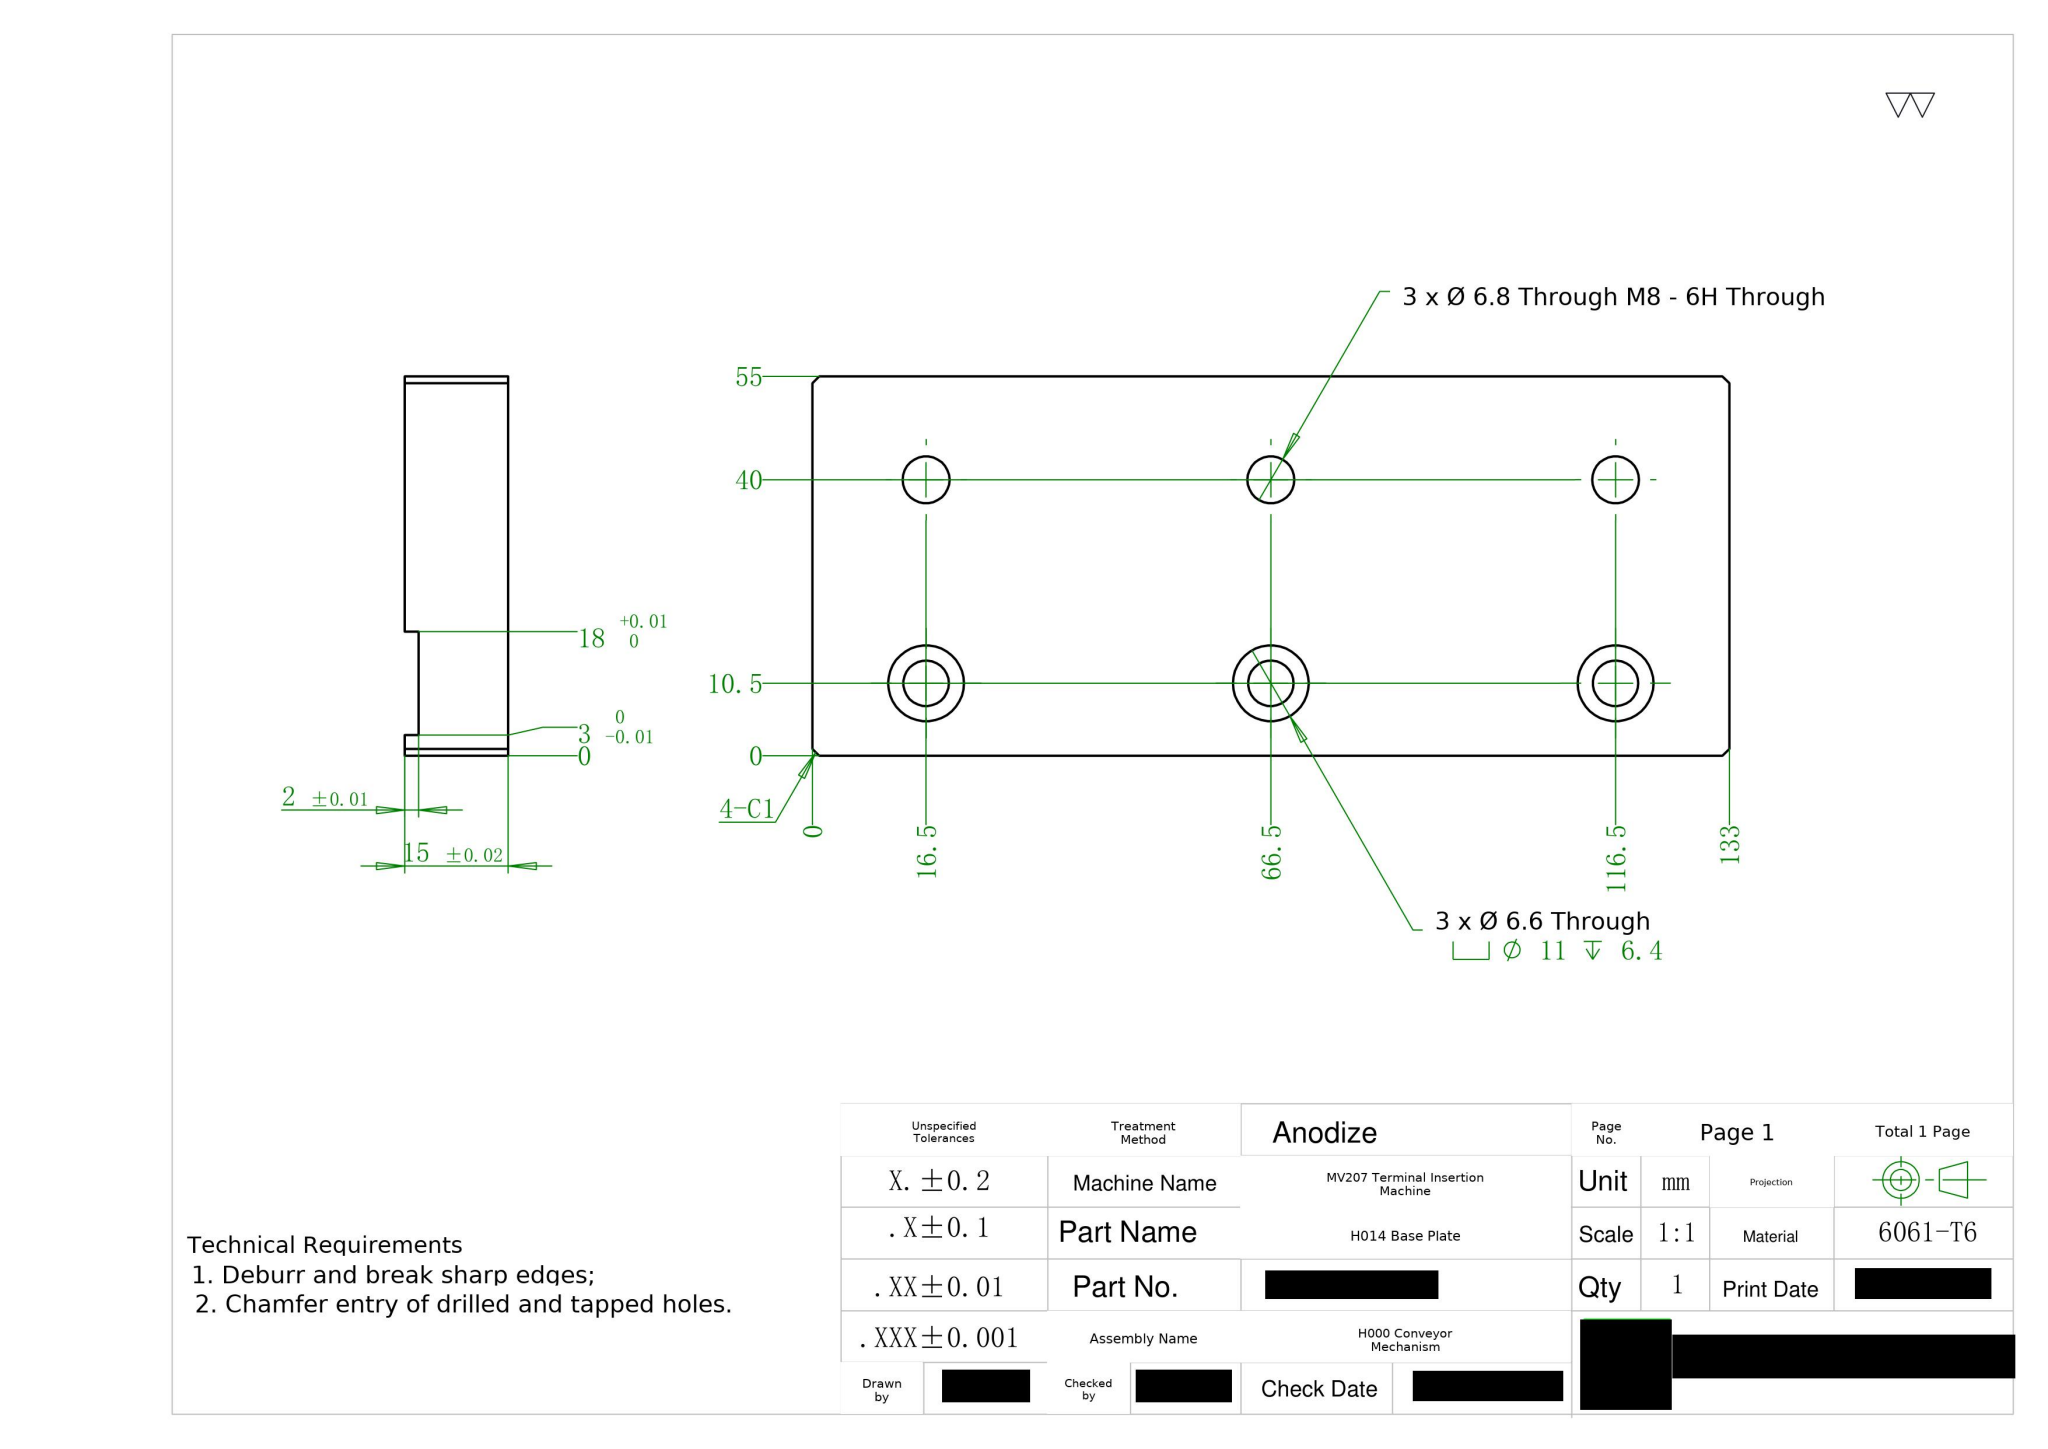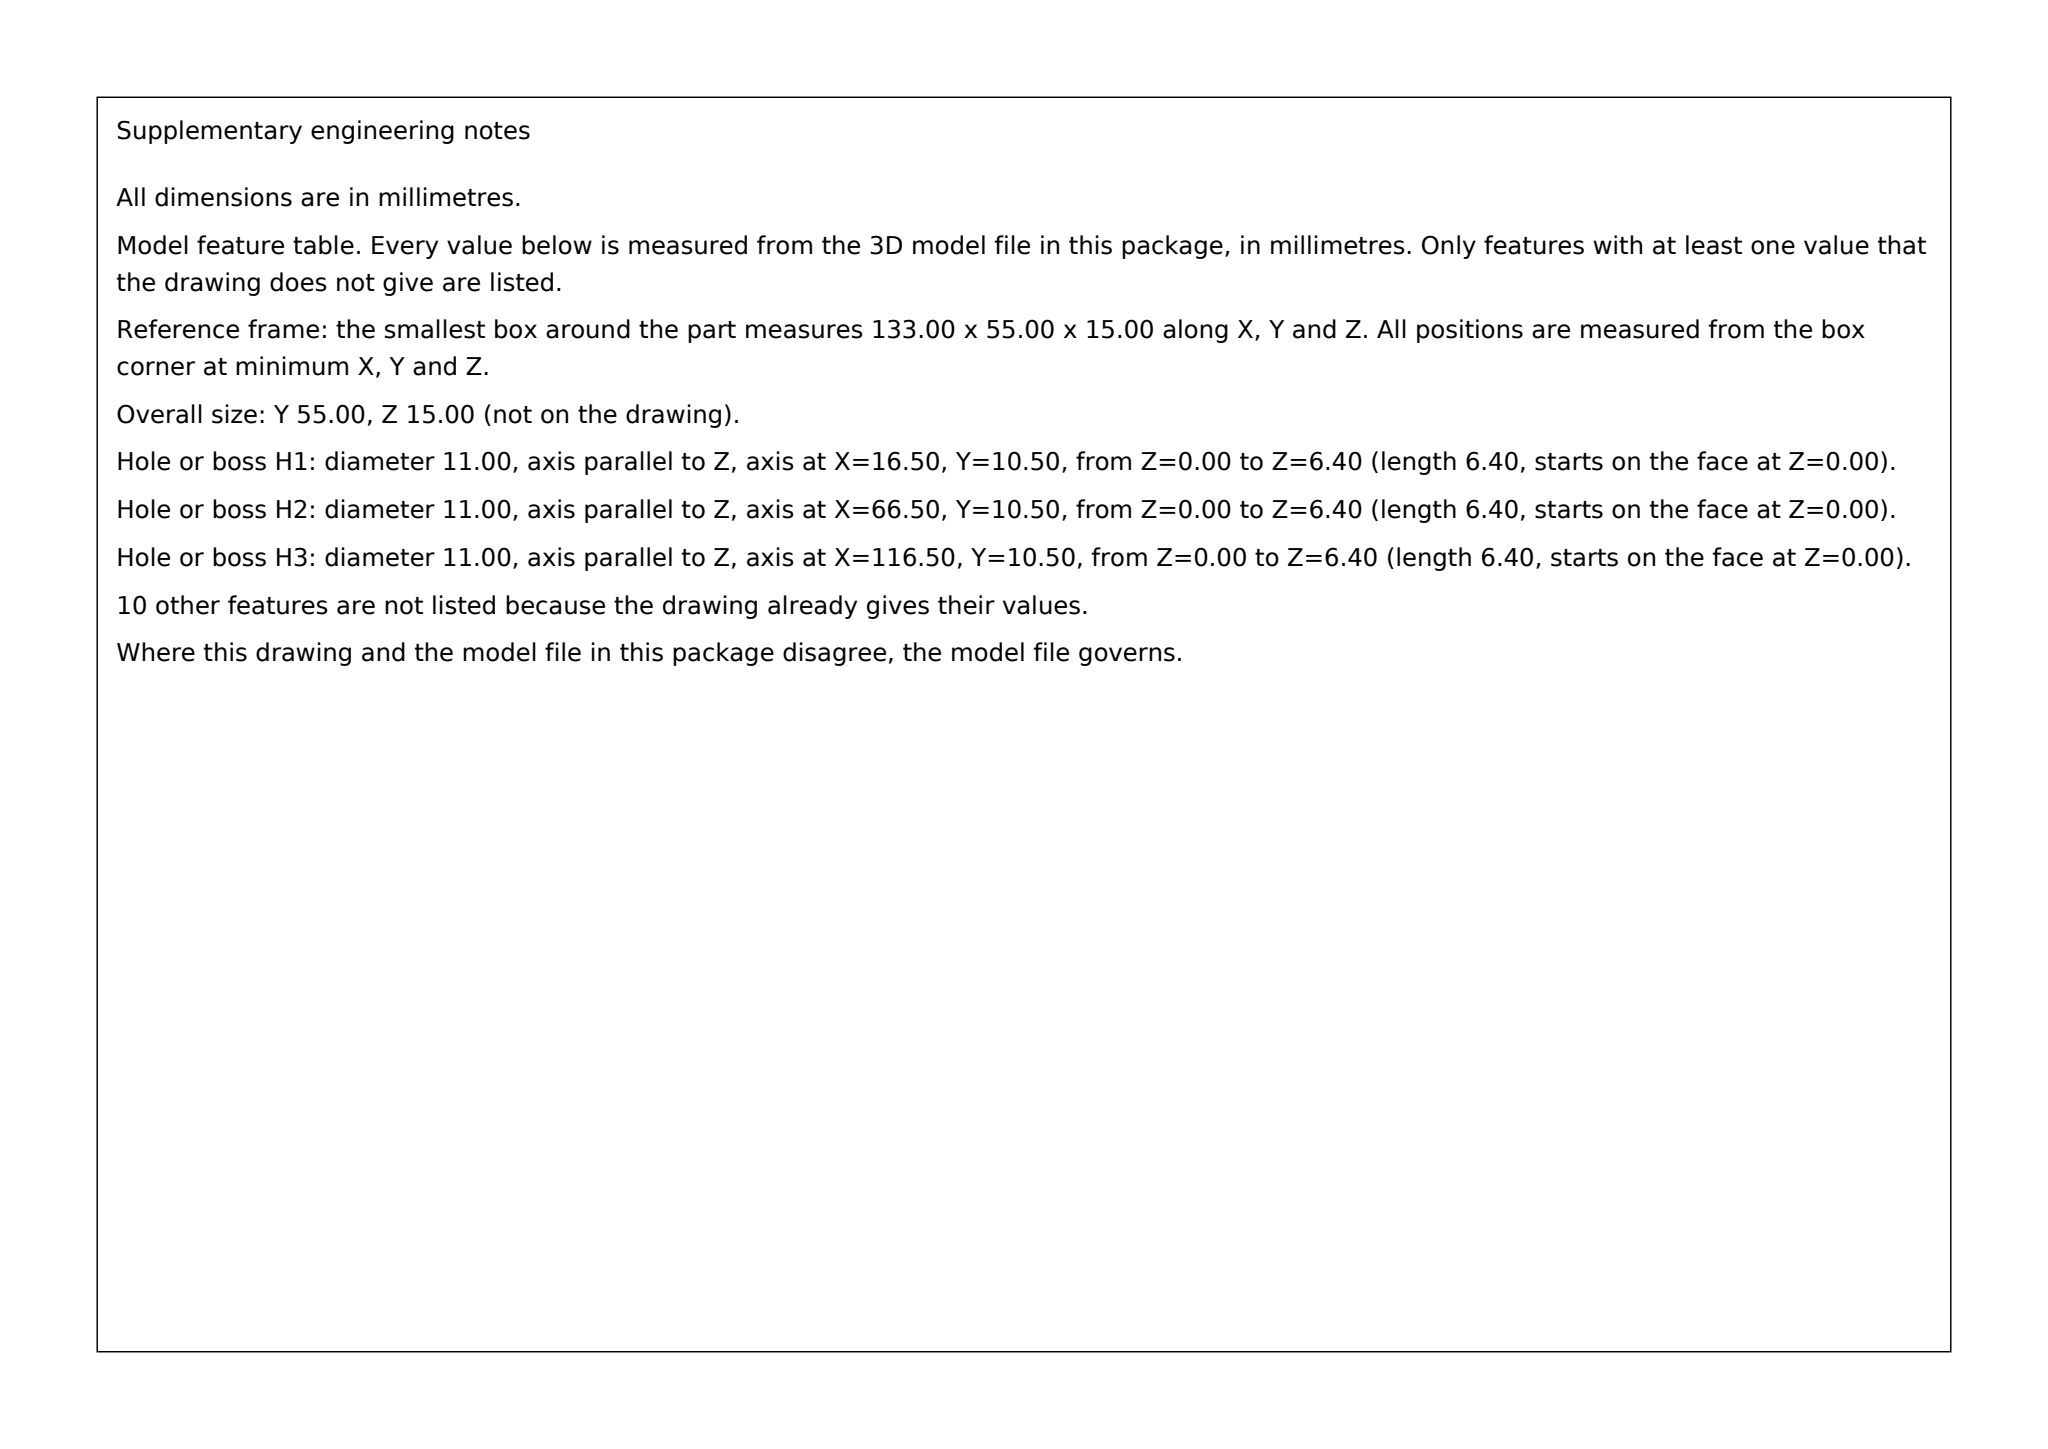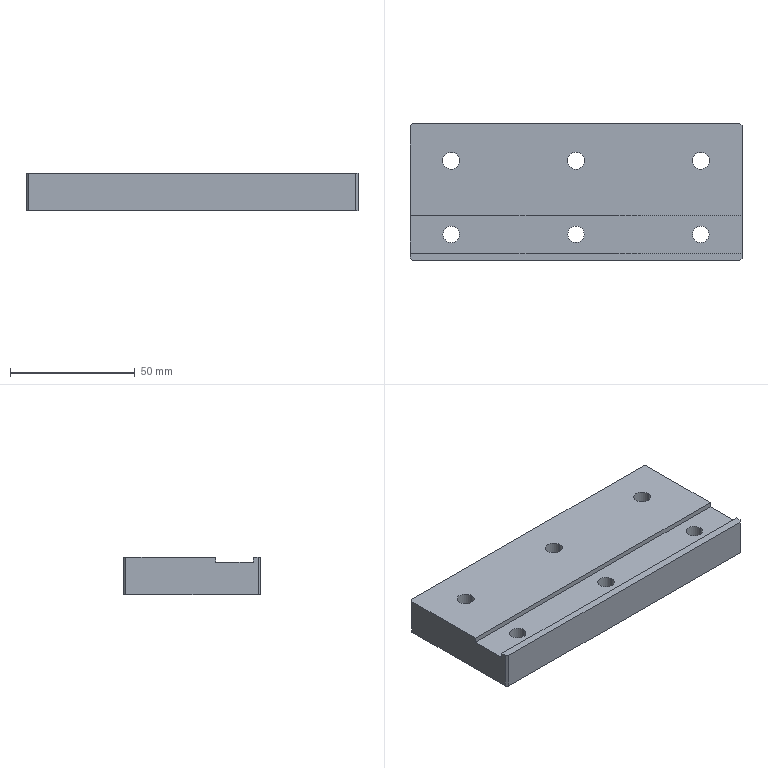Part | SolidWorks | mm | material 6061-T6 | 1 solid | 35 faces | box 133 x 55 x 15 mm | volume 101569 mm3 | cylinder 18 | plane 17 | commonest cylinder face diameters 11 x6 6.6 x6 6.8 x6
build123d program:
from build123d import *

# Parameters (mm, degrees)
SKETCH1_W                                       = 133
SKETCH1_H                                       = 55
BOSS_EXTRUDE1_DEPTH                             = 15
M8_TAPPED_HOLE1_D                               = 6.8
SKETCH9_W                                       = 2
SKETCH9_H                                       = 15
CUT_EXTRUDE2_DEPTH                              = 137.639
M6_HEX_SOCKET_HEAD_CAP_SCREW_CBORE1_D           = 6.6
M6_HEX_SOCKET_HEAD_CAP_SCREW_CBORE1_CBORE_D     = 11
M6_HEX_SOCKET_HEAD_CAP_SCREW_CBORE1_CBORE_DEPTH = 6.4
CHAMFER2_SIZE                                   = 1


with BuildPart() as part:
    # Sketch1 → Boss-Extrude1 (new body)
    with BuildSketch(Plane.XY):
        Rectangle(SKETCH1_W, SKETCH1_H)
    extrude(amount=BOSS_EXTRUDE1_DEPTH)

    # M8 Tapped Hole1 (through all)
    with Locations(Plane.XY.offset(15)):
        with Locations((-50, 12.5), (50, 12.5), (0, 12.5)):
            Hole(M8_TAPPED_HOLE1_D / 2)

    # Sketch9 → Cut-Extrude2 (cut, through all)
    with BuildSketch(Plane.ZY.offset(66.5)):
        with Locations((14, -17)):
            Rectangle(SKETCH9_W, SKETCH9_H)
    extrude(amount=-CUT_EXTRUDE2_DEPTH, mode=Mode.SUBTRACT)

    # M6 Hex Socket Head Cap Screw CBORE1 (through all)
    with Locations(Plane(origin=(0, 0, 0), x_dir=(-1, 0, 0), z_dir=(0, 0, -1))):
        with Locations((50, -17), (0, -17), (-50, -17)):
            CounterBoreHole(M6_HEX_SOCKET_HEAD_CAP_SCREW_CBORE1_D / 2, M6_HEX_SOCKET_HEAD_CAP_SCREW_CBORE1_CBORE_D / 2, M6_HEX_SOCKET_HEAD_CAP_SCREW_CBORE1_CBORE_DEPTH)

    # Chamfer2
    chamfer2_edges = [part.edges().sort_by_distance(p)[0] for p in [
        (66.5, -27.5, 7.5),
        (-66.5, -27.5, 7.5),
        (-66.5, 27.5, 7.5),
        (66.5, 27.5, 7.5),
    ]]
    chamfer(chamfer2_edges, length=CHAMFER2_SIZE)


solid = part.part